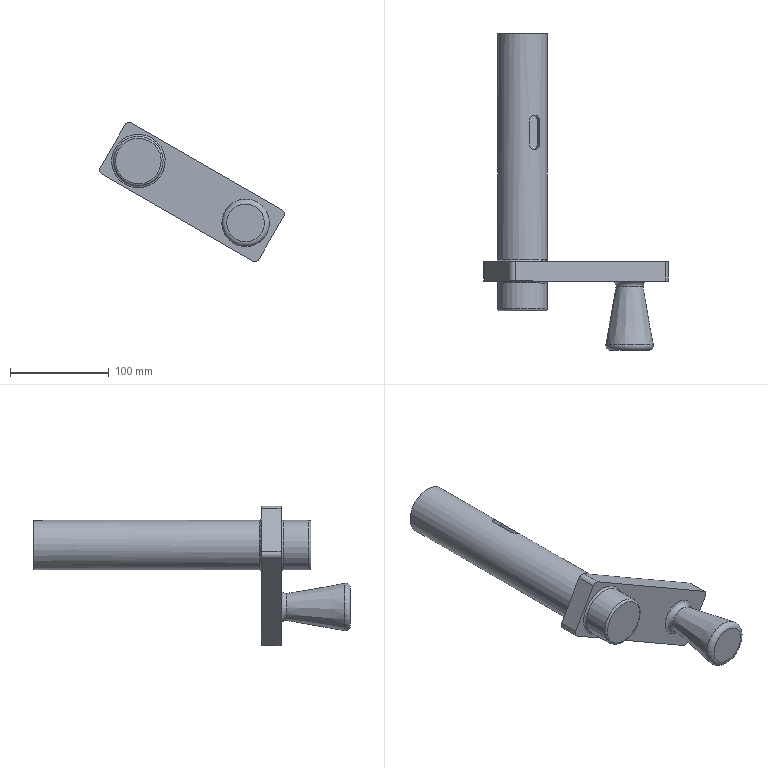Component | NX | KOL | 1 solid | 26 faces | volume 810661 mm3 | plane 12 | cylinder 8 | torus 5 | cone 1 | commonest cylinder face diameters 10 x4 50 x2 12 x2